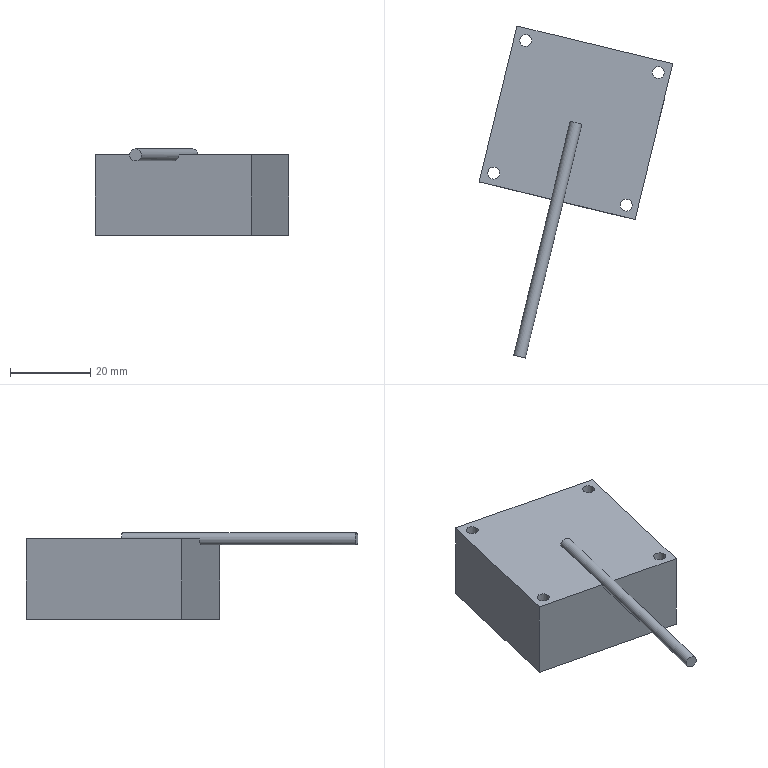Component | NX | BLOCK | 1 solid | 17 faces | volume 30402 mm3 | plane 10 | cylinder 7 | commonest cylinder face diameters 3 x5 15 x1 8 x1